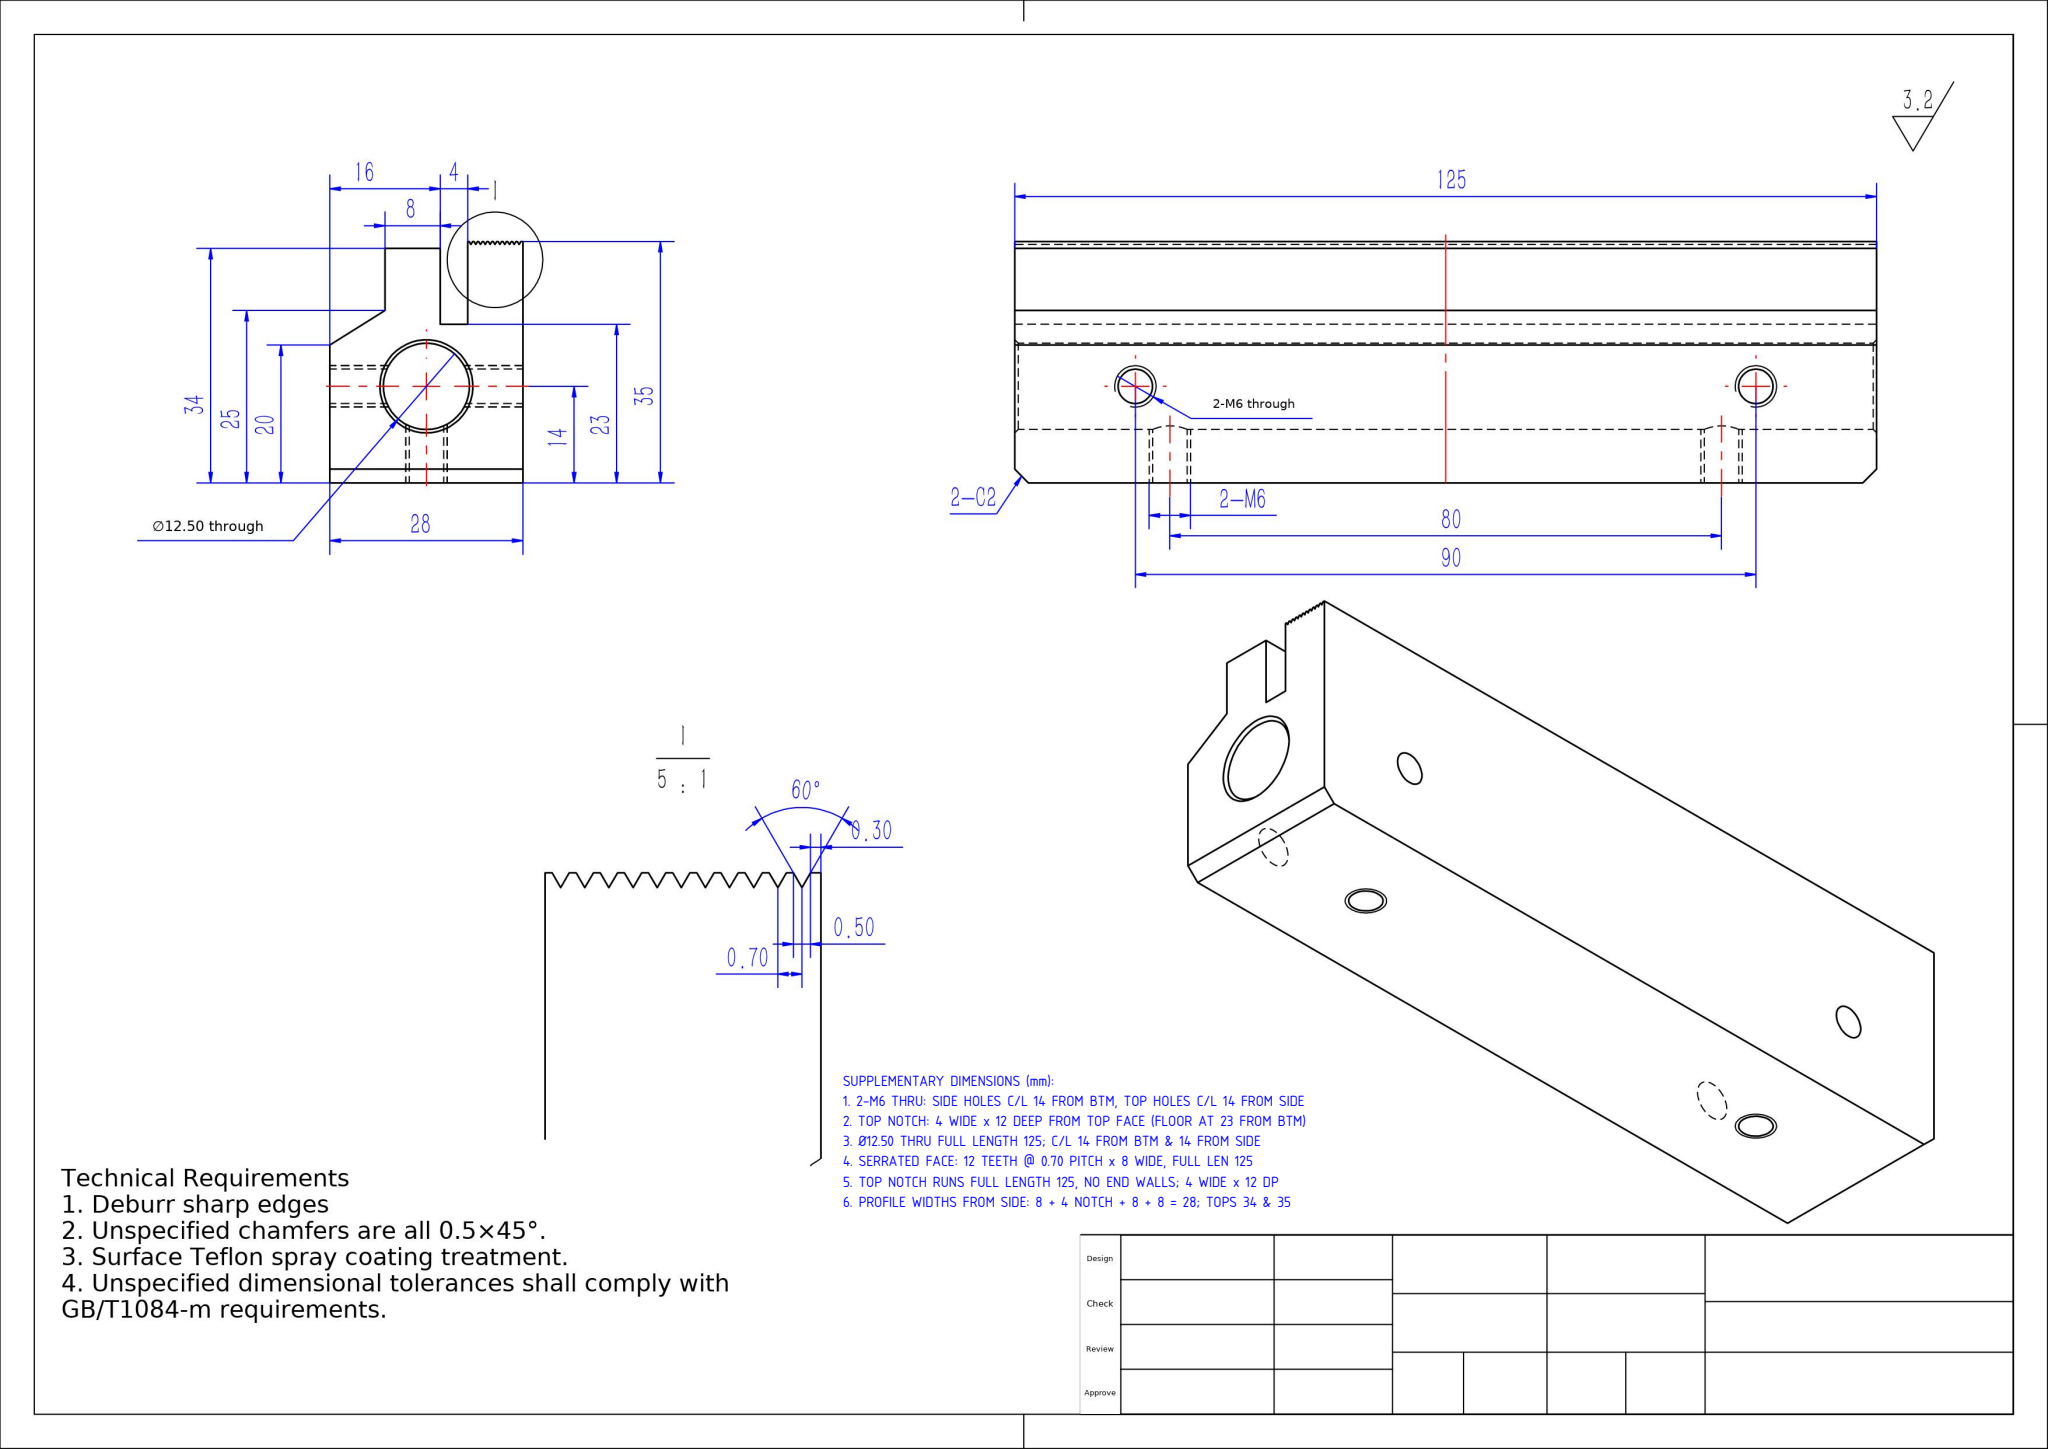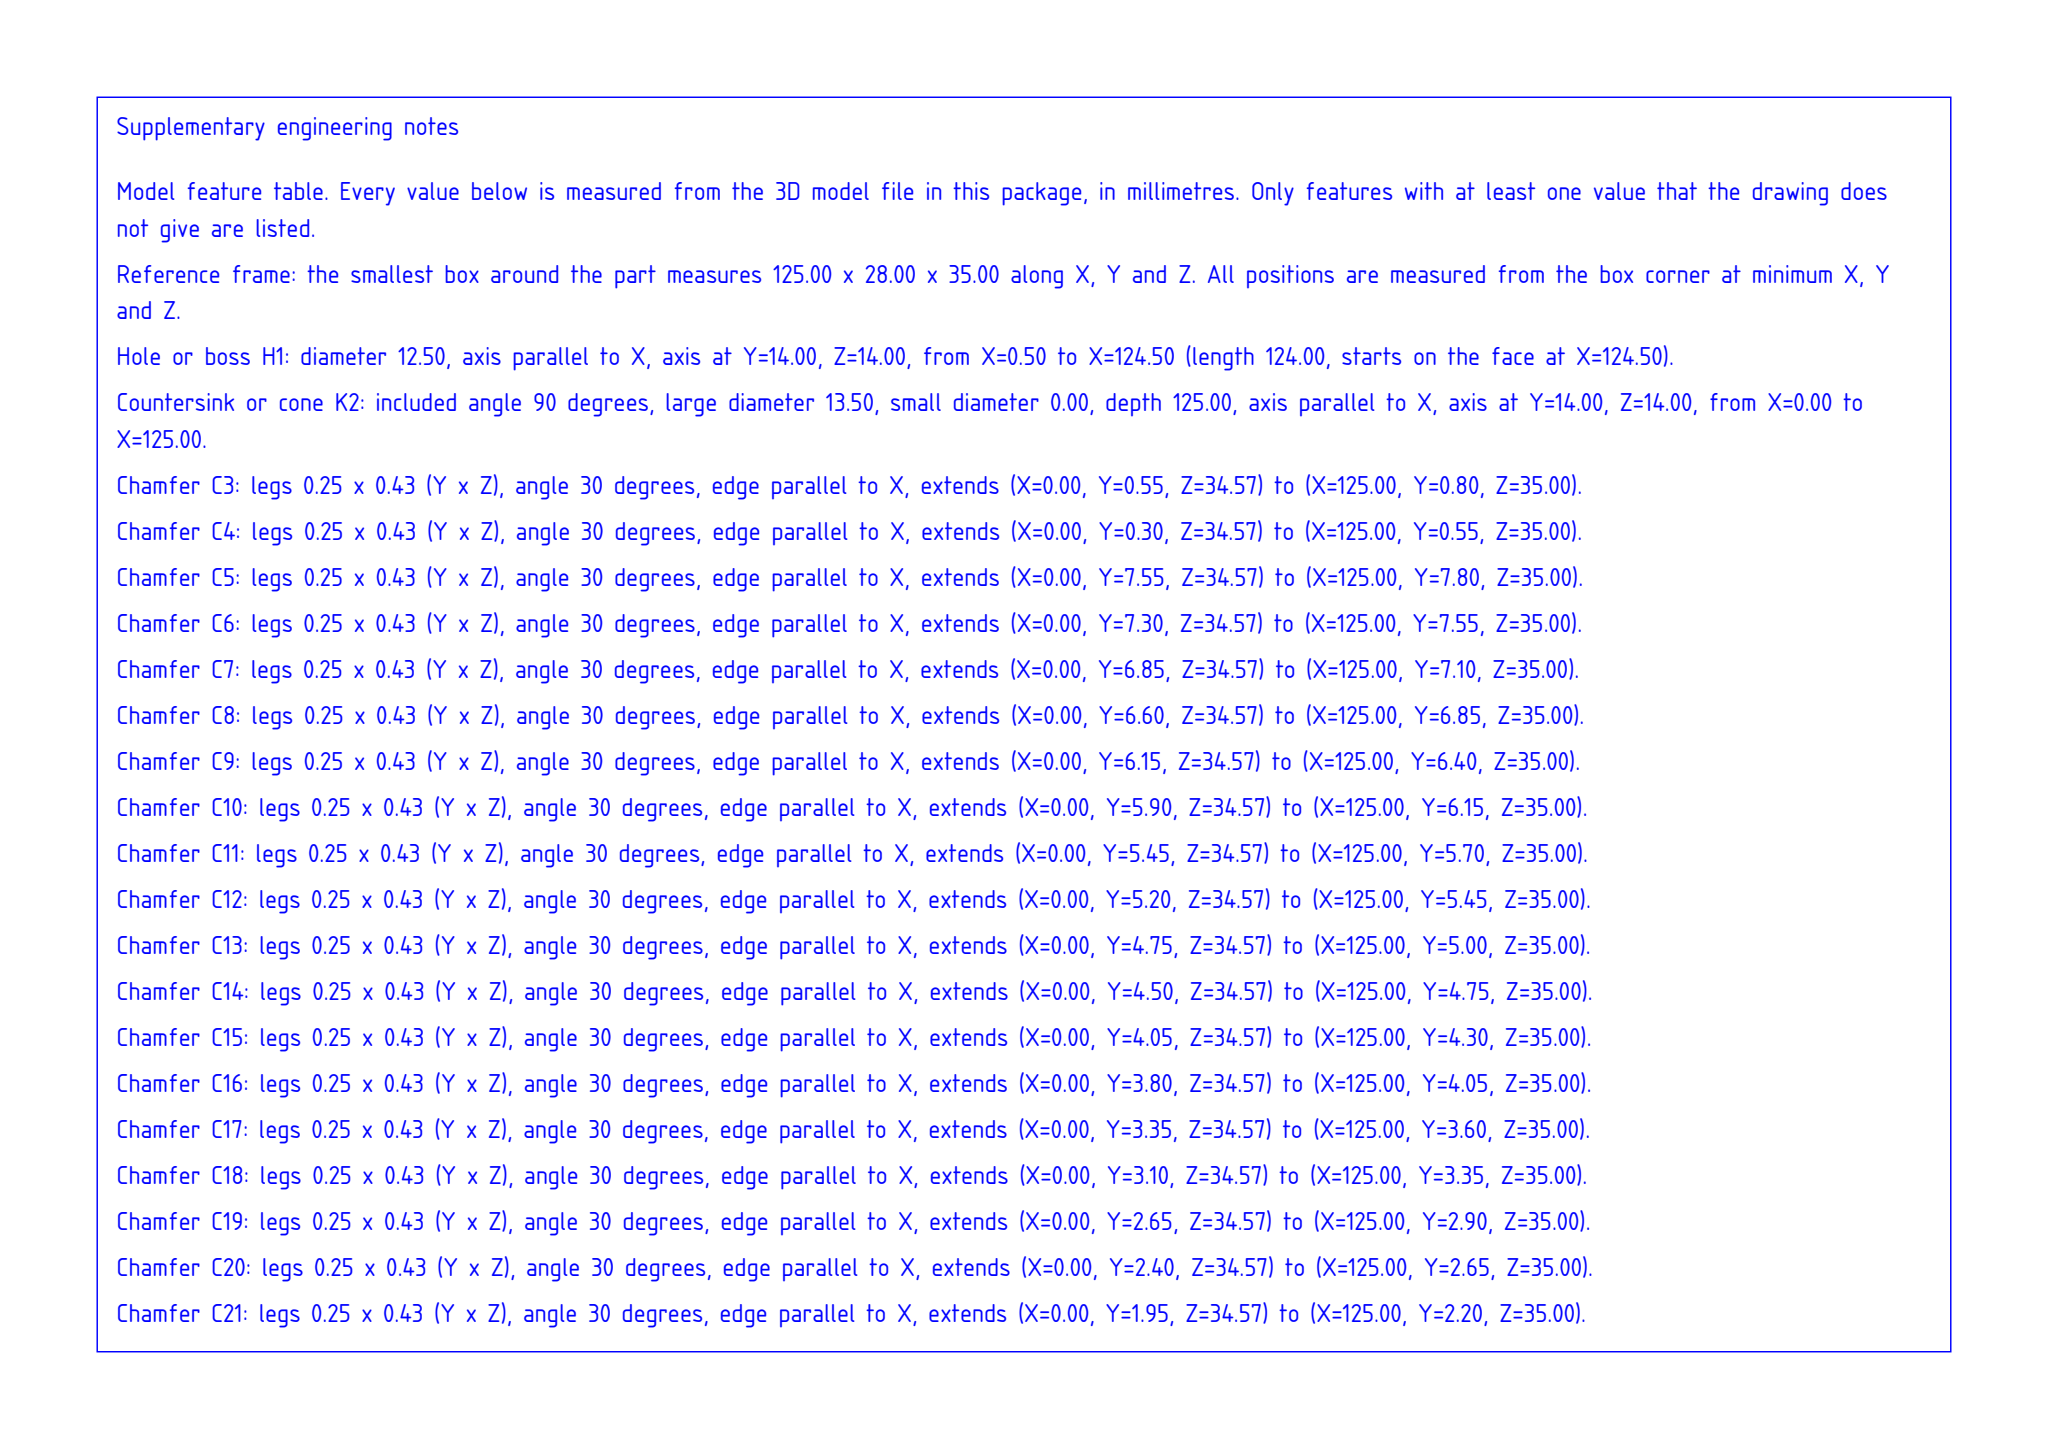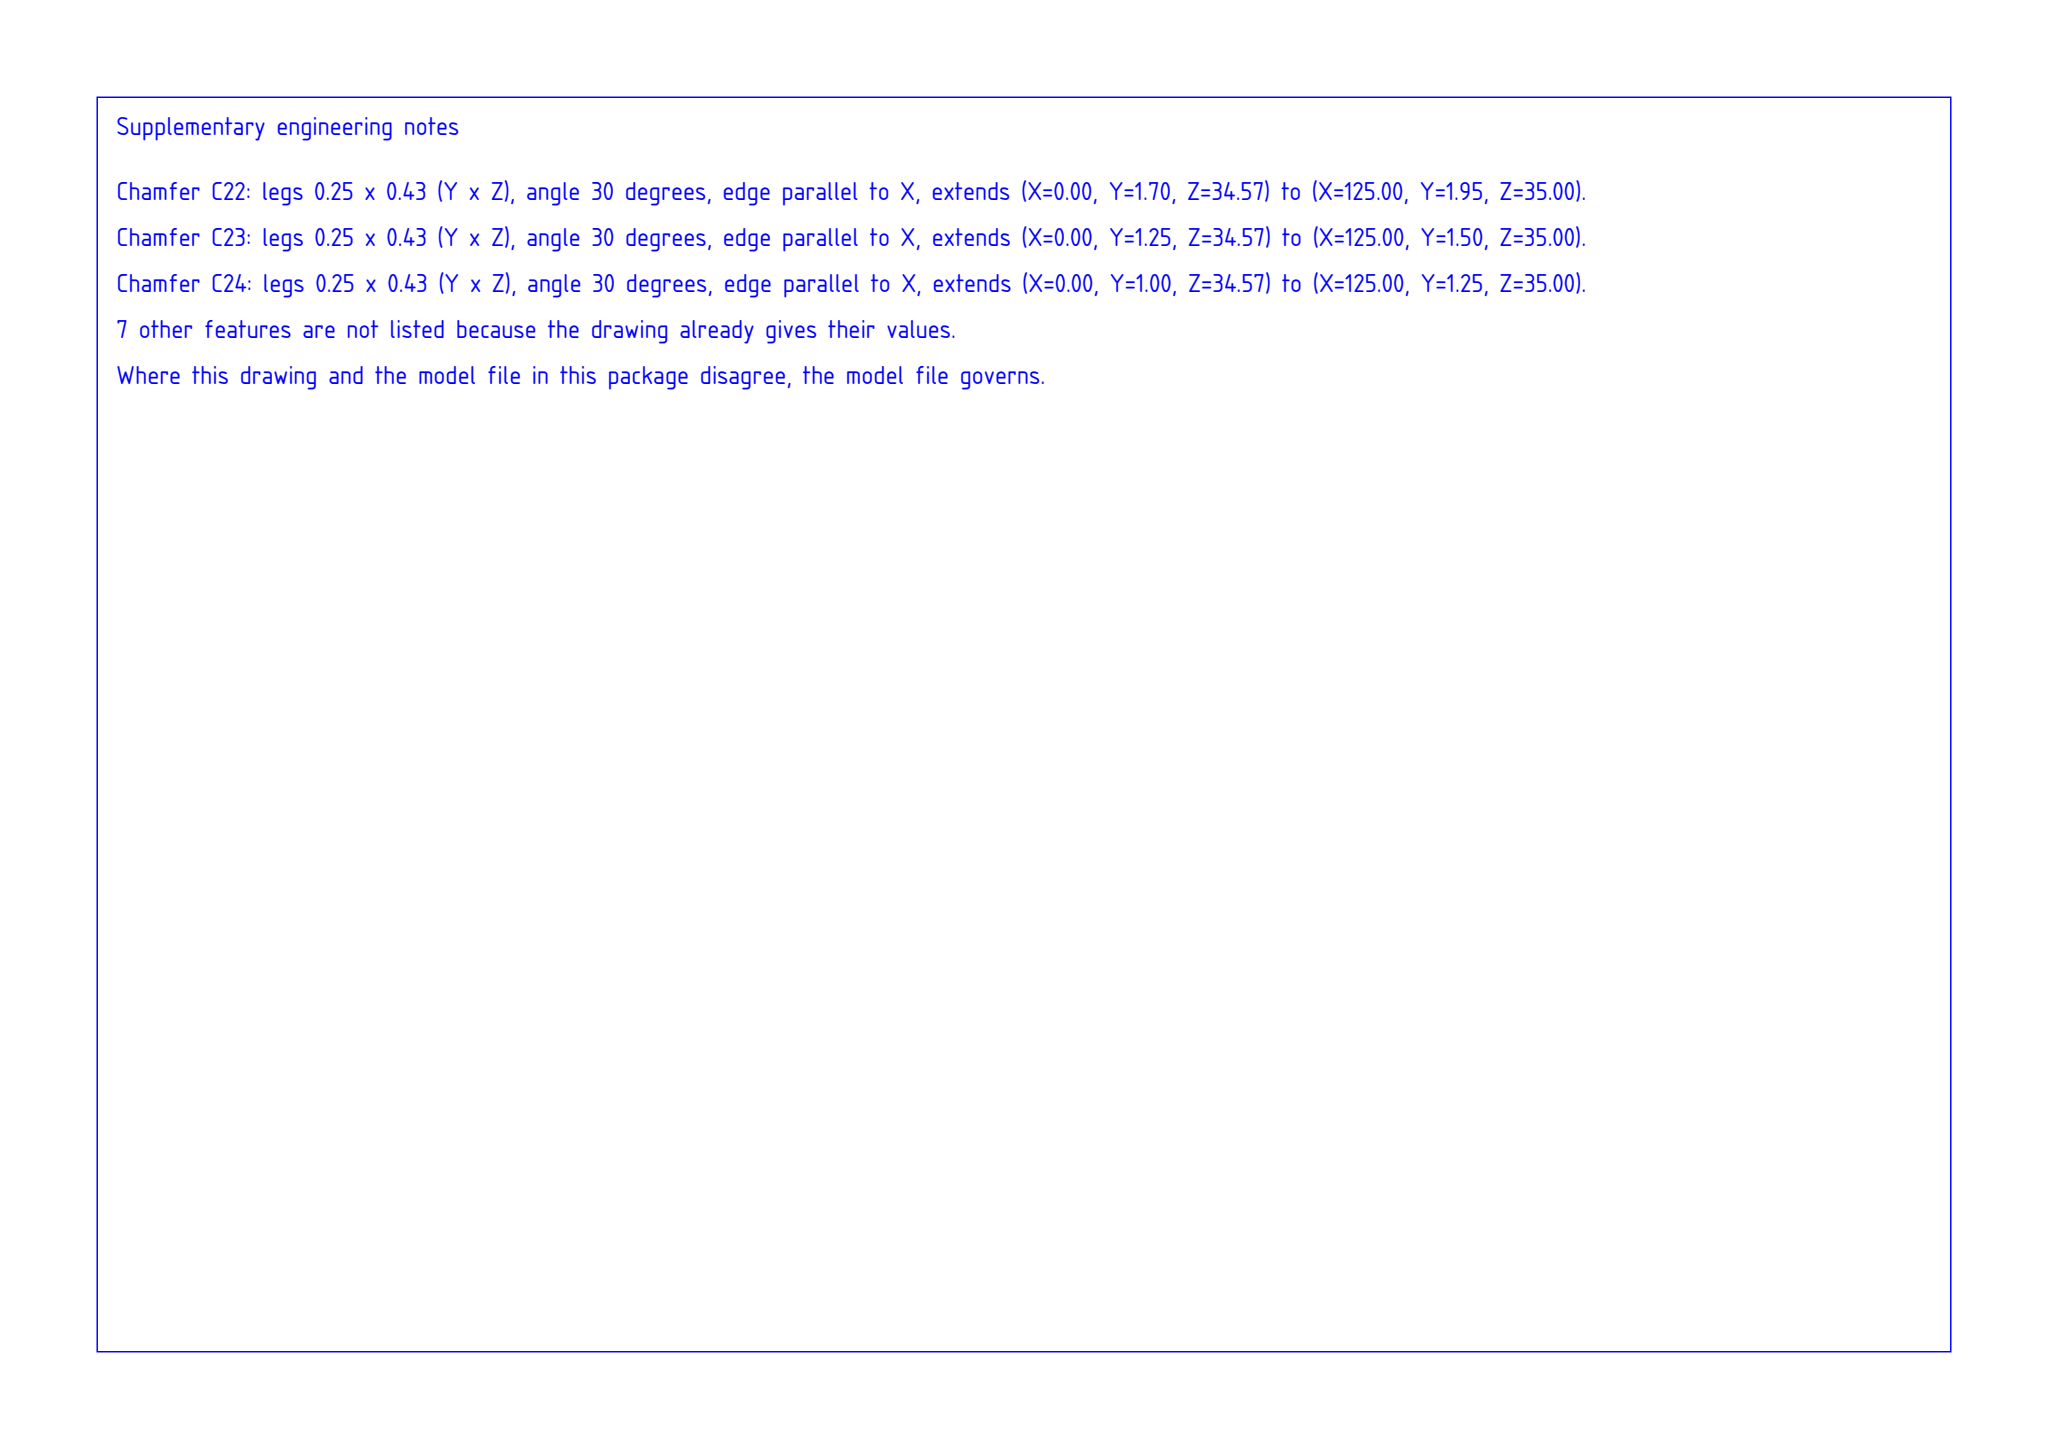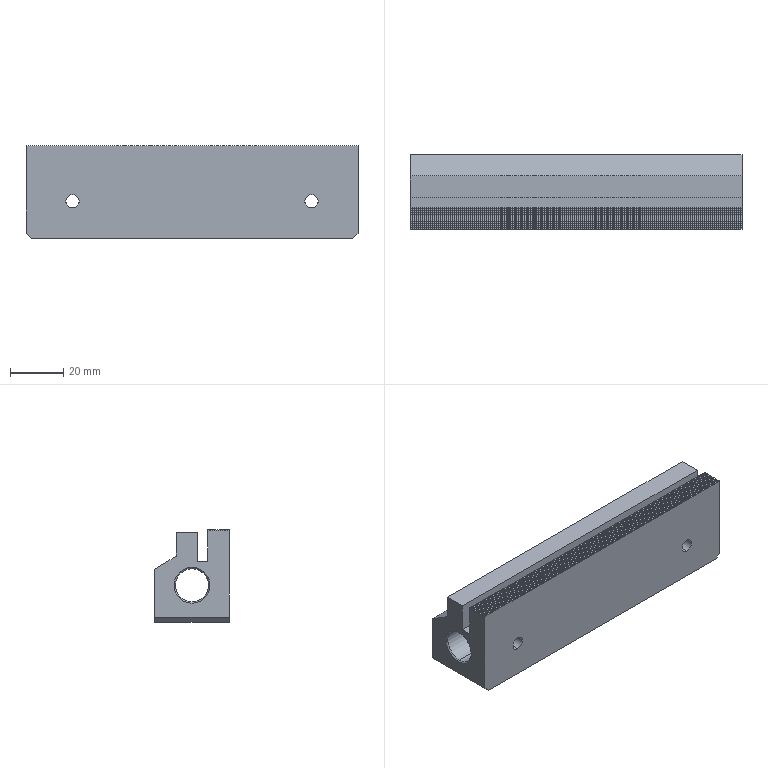Part | SolidWorks | mm | 1 solid | 65 faces | box 125 x 28 x 35 mm | volume 86461 mm3 | plane 47 | cylinder 14 | cone 4 | commonest cylinder face diameters 5 x12 12.5 x2
build123d program:
from build123d import *

# Parameters (mm, degrees)
BOSS_EXTRUDE1_DEPTH   = 62.5
SKETCH2_W             = 12
SKETCH2_H             = 4
CUT_EXTRUDE1_DEPTH    = 75
SKETCH3_R             = 6.25
CUT_EXTRUDE2_DEPTH    = 75
M6_TAPPED_HOLE1_D     = 5
M6_TAPPED_HOLE1_DEPTH = 15
M6_TAPPED_HOLE1_TIP   = 1.502
M6_TAPPED_HOLE2_D     = 5
M6_TAPPED_HOLE2_DEPTH = 33
M6_TAPPED_HOLE2_TIP   = 1.502
CUT_EXTRUDE4_DEPTH    = 133.793
LPATTERN2_COUNT       = 11
LPATTERN2_PITCH       = 0.7
CHAMFER1_SIZE         = 2
CHAMFER2_SIZE         = 0.5
SKETCH11_W            = 1
SKETCH11_H            = 8
CUT_EXTRUDE5_DEPTH    = 133.793


with BuildPart() as part:
    # Sketch1 → Boss-Extrude1 (new, symmetric)
    with BuildSketch(Plane(origin=(0, 0, 0), x_dir=(0, 1, 0), z_dir=(-1, 0, 0))):
        Polygon((20, -35), (20, -25), (28, -20), (28, 0), (0, 0), (0, -35), align=None)
    extrude(amount=BOSS_EXTRUDE1_DEPTH, both=True)

    # Sketch2 → Cut-Extrude1 (cut, symmetric)
    with BuildSketch(Plane(origin=(0, 0, 0), x_dir=(0, 0, -1), z_dir=(1, 0, 0))):
        with Locations((-29, 10)):
            Rectangle(SKETCH2_W, SKETCH2_H)
    extrude(amount=CUT_EXTRUDE1_DEPTH, both=True, mode=Mode.SUBTRACT)

    # Sketch3 → Cut-Extrude2 (cut, symmetric)
    with BuildSketch(Plane(origin=(0, 0, 0), x_dir=(0, 0, -1), z_dir=(1, 0, 0))):
        with Locations((-14, 14)):
            Circle(SKETCH3_R)
    extrude(amount=CUT_EXTRUDE2_DEPTH, both=True, mode=Mode.SUBTRACT)

    # M6 Tapped Hole1
    with Locations(Plane(origin=(0, 0, 0), x_dir=(-1, 0, 0), z_dir=(0, 0, -1))):
        with Locations((-40, 14), (40, 14)):
            Hole(M6_TAPPED_HOLE1_D / 2, depth=M6_TAPPED_HOLE1_DEPTH)
            with Locations((0, 0, -(M6_TAPPED_HOLE1_DEPTH + M6_TAPPED_HOLE1_TIP / 2))):  # 118° drill point
                Cone(0, M6_TAPPED_HOLE1_D / 2, M6_TAPPED_HOLE1_TIP, mode=Mode.SUBTRACT)

    # M6 Tapped Hole2
    with Locations(Plane(origin=(0, 28, 0), x_dir=(-1, 0, 0), z_dir=(0, 1, 0))):
        with Locations((45, 14), (-45, 14)):
            Hole(M6_TAPPED_HOLE2_D / 2, depth=M6_TAPPED_HOLE2_DEPTH)
            with Locations((0, 0, -(M6_TAPPED_HOLE2_DEPTH + M6_TAPPED_HOLE2_TIP / 2))):  # 118° drill point
                Cone(0, M6_TAPPED_HOLE2_D / 2, M6_TAPPED_HOLE2_TIP, mode=Mode.SUBTRACT)

    # Sketch10 → Cut-Extrude4 (cut, through all)
    with BuildSketch(Plane.ZY.offset(62.5)):
        Polygon((35, 0.8), (35, 0.3), (34.567, 0.55), align=None)
    cut_extrude4 = extrude(amount=-CUT_EXTRUDE4_DEPTH, mode=Mode.SUBTRACT)

    # LPattern2: Cut-Extrude4 ×11
    with Locations(*[(0, i * LPATTERN2_PITCH, 0) for i in range(1, LPATTERN2_COUNT)]):
        add(cut_extrude4, mode=Mode.SUBTRACT)

    # Chamfer1
    chamfer1_edges = [part.edges().sort_by_distance(p)[0] for p in [
        (-62.5, 14, 0),
        (62.5, 14, 0),
    ]]
    chamfer(chamfer1_edges, length=CHAMFER1_SIZE)

    # Chamfer2
    chamfer2_edges = [part.edges().sort_by_distance(p)[0] for p in [
        (-62.5, 14, 20.25),
        (62.5, 14, 20.25),
    ]]
    chamfer(chamfer2_edges, length=CHAMFER2_SIZE)

    # Sketch11 → Cut-Extrude5 (cut, through all)
    with BuildSketch(Plane.ZY.offset(62.5)):
        with Locations((34.5, 16)):
            Rectangle(SKETCH11_W, SKETCH11_H)
    extrude(amount=-CUT_EXTRUDE5_DEPTH, mode=Mode.SUBTRACT)


solid = part.part